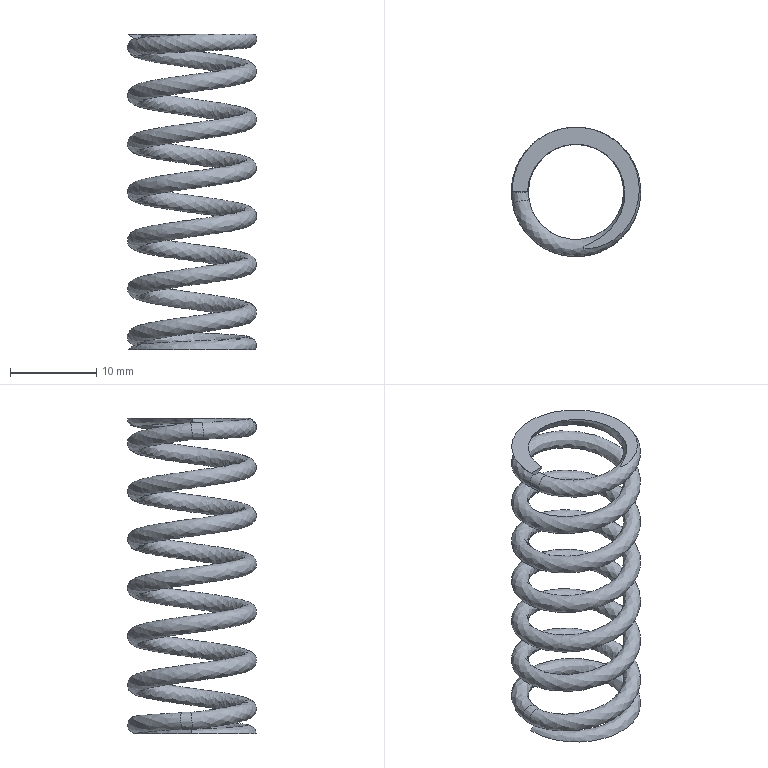Component | NX | SPRING | 1 solid | 9 faces | volume 949 mm3 | spline 5 | plane 4